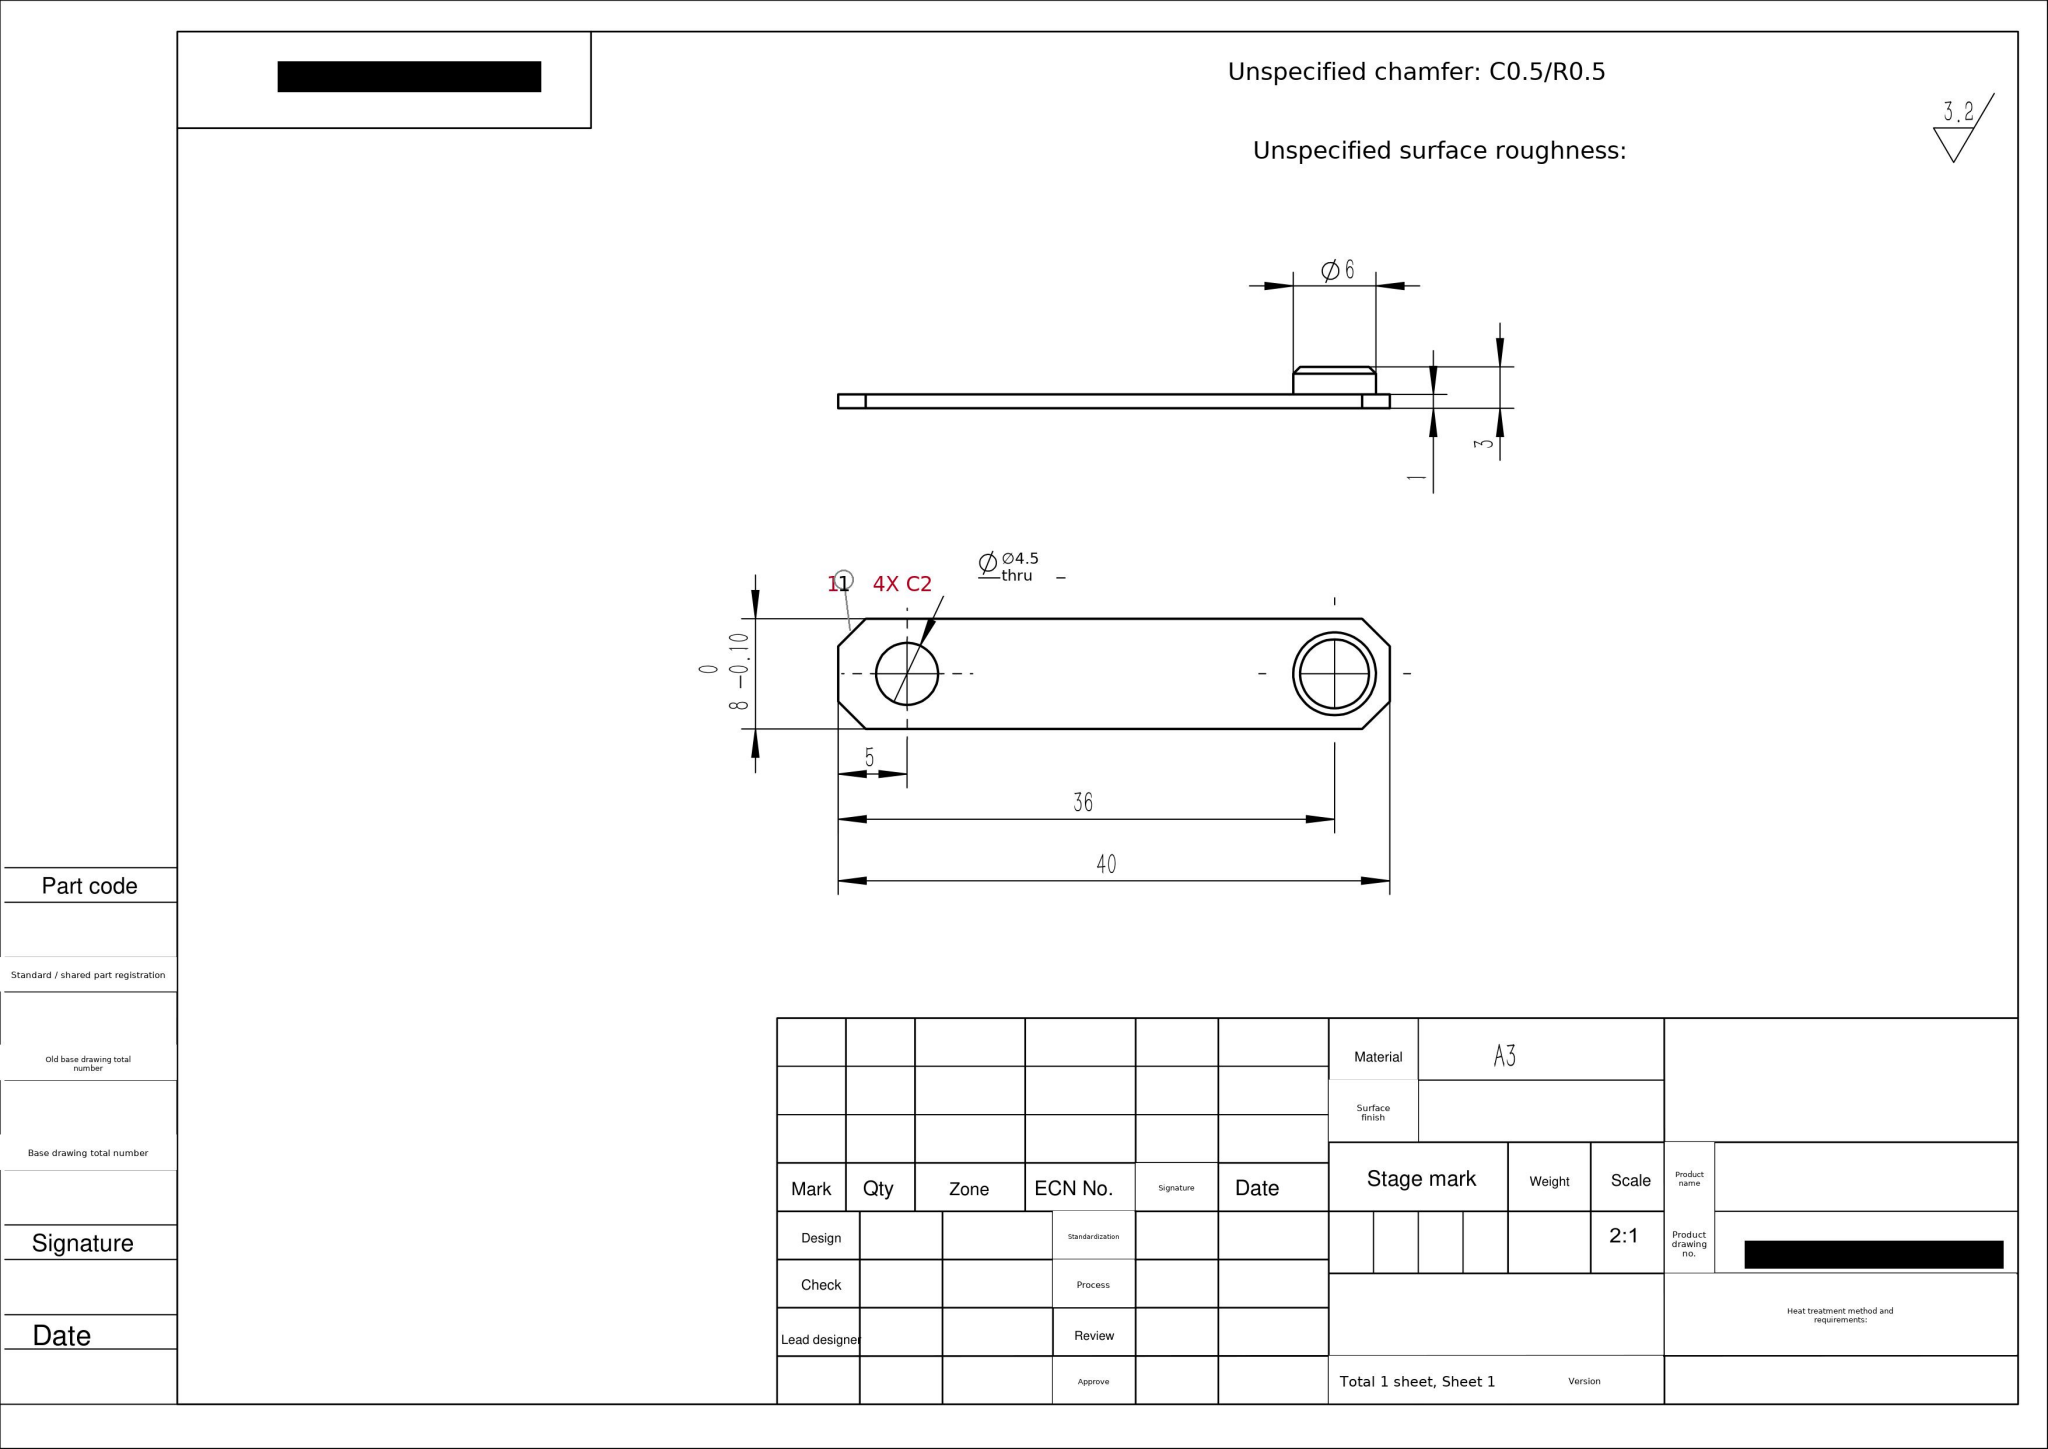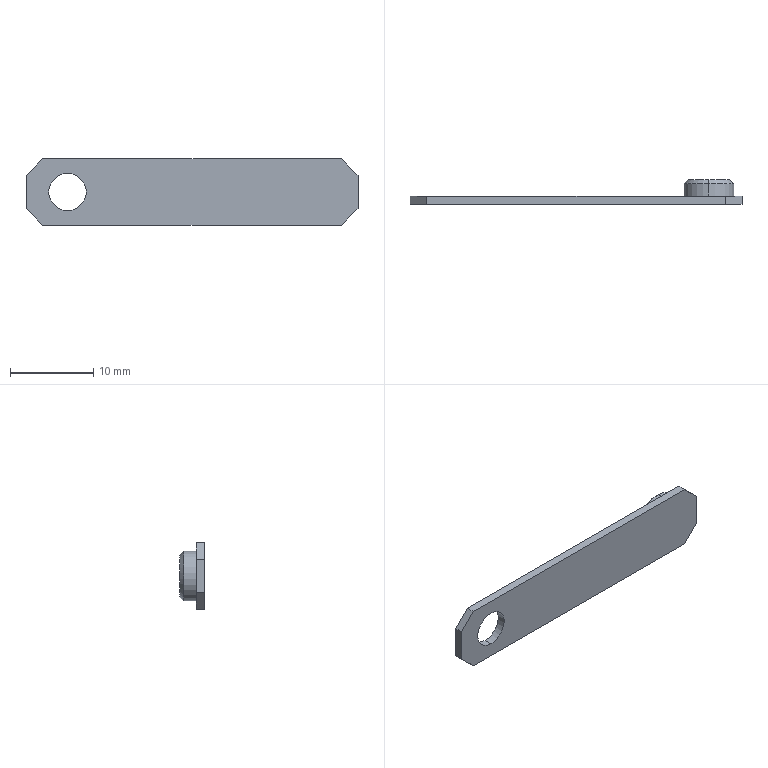Part | SolidWorks | mm | material A3 | 1 solid | 17 faces | box 40 x 3 x 8 mm | volume 350 mm3 | plane 11 | cylinder 4 | cone 2 | commonest cylinder face diameters 4.5 x2 6 x2
build123d program:
from build123d import *

# Parameters (mm, degrees)
SKETCH1_W           = 40
SKETCH1_H           = 8
BOSS_EXTRUDE1_DEPTH = 2
SKETCH2_R           = 2.25
CUT_EXTRUDE1_DEPTH  = 32.281
SKETCH3_R           = 3
BOSS_EXTRUDE2_DEPTH = 1
CHAMFER1_SIZE       = 0.5
CUT_EXTRUDE2_START  = -1
SKETCH4_W           = 49.789
SKETCH4_H           = 17.489
SKETCH4_R           = 3
CUT_EXTRUDE2_DEPTH  = 1
CHAMFER2_SIZE       = 2


with BuildPart() as part:
    # Sketch1 → Boss-Extrude1 (new body)
    with BuildSketch(Plane(origin=(0, 0, 0), x_dir=(1, 0, 0), z_dir=(0, 1, 0))):
        with Locations((10.307, 3.484)):
            Rectangle(SKETCH1_W, SKETCH1_H)
    extrude(amount=BOSS_EXTRUDE1_DEPTH)

    # Sketch2 → Cut-Extrude1 (cut, through all)
    with BuildSketch(Plane(origin=(0, 2, 0), x_dir=(1, 0, 0), z_dir=(0, 1, 0))):
        with Locations(Location((-4.693, 3.484, 0), (0, 0, 270))):
            Circle(SKETCH2_R)
    extrude(amount=-CUT_EXTRUDE1_DEPTH, mode=Mode.SUBTRACT)

    # Sketch3 → Boss-Extrude2 (add)
    with BuildSketch(Plane(origin=(0, 2, 0), x_dir=(1, 0, 0), z_dir=(0, 1, 0))):
        with Locations(Location((26.307, 3.484, 0), (0, 0, 270))):
            Circle(SKETCH3_R)
    extrude(amount=BOSS_EXTRUDE2_DEPTH)

    # Chamfer1
    chamfer1_edges = [part.edges().sort_by_distance(p)[0] for p in [
        (26.307, 3, -6.484),
    ]]
    chamfer(chamfer1_edges, length=CHAMFER1_SIZE)

    # Sketch4 → Cut-Extrude2 (cut)
    with BuildSketch(Plane(origin=(0, 2, 0), x_dir=(1, 0, 0), z_dir=(0, 1, 0)).offset(CUT_EXTRUDE2_START)):
        with Locations((15.201, 2.858)):
            Rectangle(SKETCH4_W, SKETCH4_H)
        with Locations(Location((26.307, 3.484, 0), (0, 0, 270))):
            Circle(SKETCH4_R, mode=Mode.SUBTRACT)
    extrude(amount=CUT_EXTRUDE2_DEPTH, mode=Mode.SUBTRACT)

    # Chamfer2
    chamfer2_edges = [part.edges().sort_by_distance(p)[0] for p in [
        (-9.693, 0.5, -7.484),
        (30.307, 0.5, -7.484),
        (30.307, 0.5, 0.5156),
        (-9.693, 0.5, 0.5156),
    ]]
    chamfer(chamfer2_edges, length=CHAMFER2_SIZE)


solid = part.part
STEP:
#1=CARTESIAN_POINT('',(-4.693,0.,-5.734));
#2=VERTEX_POINT('',#1);
#3=CARTESIAN_POINT('',(-4.693,0.,-1.234));
#4=VERTEX_POINT('',#3);
#5=CARTESIAN_POINT('',(-4.693,0.,-3.484));
#6=DIRECTION('',(0.,1.,0.));
#7=DIRECTION('',(0.,0.,1.));
#8=AXIS2_PLACEMENT_3D('',#5,#6,#7);
#9=CIRCLE('',#8,2.25);
#10=EDGE_CURVE('',#2,#4,#9,.T.);
#11=ORIENTED_EDGE('',*,*,#10,.F.);
#12=CARTESIAN_POINT('',(-4.693,1.,-5.734));
#13=VERTEX_POINT('',#12);
#14=CARTESIAN_POINT('',(-4.693,0.,-5.734));
#15=DIRECTION('',(0.,1.,0.));
#16=VECTOR('',#15,1000.);
#17=LINE('',#14,#16);
#18=EDGE_CURVE('',#2,#13,#17,.T.);
#19=ORIENTED_EDGE('',*,*,#18,.T.);
#20=CARTESIAN_POINT('',(-4.693,1.,-1.234));
#21=VERTEX_POINT('',#20);
#22=CARTESIAN_POINT('',(-4.693,1.,-3.484));
#23=DIRECTION('',(0.,-1.,0.));
#24=DIRECTION('',(0.,0.,1.));
#25=AXIS2_PLACEMENT_3D('',#22,#23,#24);
#26=CIRCLE('',#25,2.25);
#27=EDGE_CURVE('',#21,#13,#26,.T.);
#28=ORIENTED_EDGE('',*,*,#27,.F.);
#29=CARTESIAN_POINT('',(-4.693,0.,-1.234));
#30=DIRECTION('',(0.,1.,0.));
#31=VECTOR('',#30,1000.);
#32=LINE('',#29,#31);
#33=EDGE_CURVE('',#4,#21,#32,.T.);
#34=ORIENTED_EDGE('',*,*,#33,.F.);
#35=EDGE_LOOP('',(#11,#19,#28,#34));
#36=FACE_OUTER_BOUND('',#35,.T.);
#37=CARTESIAN_POINT('',(-4.693,0.,-3.484));
#38=DIRECTION('',(0.,1.,0.));
#39=DIRECTION('',(0.,0.,1.));
#40=AXIS2_PLACEMENT_3D('',#37,#38,#39);
#41=CYLINDRICAL_SURFACE('',#40,2.25);
#42=ADVANCED_FACE('',(#36),#41,.F.);
#43=CARTESIAN_POINT('',(26.307,3.,-0.9844));
#44=VERTEX_POINT('',#43);
#45=CARTESIAN_POINT('',(26.307,3.,-5.984));
#46=VERTEX_POINT('',#45);
#47=CARTESIAN_POINT('',(26.307,3.,-3.484));
#48=DIRECTION('',(0.,1.,0.));
#49=DIRECTION('',(0.,0.,1.));
#50=AXIS2_PLACEMENT_3D('',#47,#48,#49);
#51=CIRCLE('',#50,2.5);
#52=EDGE_CURVE('',#44,#46,#51,.T.);
#53=ORIENTED_EDGE('',*,*,#52,.F.);
#54=CARTESIAN_POINT('',(26.307,2.5,-0.4844));
#55=VERTEX_POINT('',#54);
#56=CARTESIAN_POINT('',(26.307,3.,-0.9844));
#57=DIRECTION('',(0.,-0.7071,0.7071));
#58=VECTOR('',#57,1000.);
#59=LINE('',#56,#58);
#60=EDGE_CURVE('',#44,#55,#59,.T.);
#61=ORIENTED_EDGE('',*,*,#60,.T.);
#62=CARTESIAN_POINT('',(26.307,2.5,-6.484));
#63=VERTEX_POINT('',#62);
#64=CARTESIAN_POINT('',(26.307,2.5,-3.484));
#65=DIRECTION('',(0.,-1.,0.));
#66=DIRECTION('',(0.,0.,1.));
#67=AXIS2_PLACEMENT_3D('',#64,#65,#66);
#68=CIRCLE('',#67,3.);
#69=EDGE_CURVE('',#63,#55,#68,.T.);
#70=ORIENTED_EDGE('',*,*,#69,.F.);
#71=CARTESIAN_POINT('',(26.307,3.,-5.984));
#72=DIRECTION('',(0.,-0.7071,-0.7071));
#73=VECTOR('',#72,1000.);
#74=LINE('',#71,#73);
#75=EDGE_CURVE('',#46,#63,#74,.T.);
#76=ORIENTED_EDGE('',*,*,#75,.F.);
#77=EDGE_LOOP('',(#53,#61,#70,#76));
#78=FACE_OUTER_BOUND('',#77,.T.);
#79=CARTESIAN_POINT('',(26.307,3.,-3.484));
#80=DIRECTION('',(0.,-1.,0.));
#81=DIRECTION('',(0.,0.,-1.));
#82=AXIS2_PLACEMENT_3D('',#79,#80,#81);
#83=CONICAL_SURFACE('',#82,2.5,0.7854);
#84=ADVANCED_FACE('',(#78),#83,.T.);
#85=ORIENTED_EDGE('',*,*,#69,.T.);
#86=CARTESIAN_POINT('',(26.307,1.,-0.4844));
#87=VERTEX_POINT('',#86);
#88=CARTESIAN_POINT('',(26.307,3.,-0.4844));
#89=DIRECTION('',(0.,-1.,0.));
#90=VECTOR('',#89,1000.);
#91=LINE('',#88,#90);
#92=EDGE_CURVE('',#55,#87,#91,.T.);
#93=ORIENTED_EDGE('',*,*,#92,.T.);
#94=CARTESIAN_POINT('',(26.307,1.,-6.484));
#95=VERTEX_POINT('',#94);
#96=CARTESIAN_POINT('',(26.307,1.,-3.484));
#97=DIRECTION('',(0.,1.,0.));
#98=DIRECTION('',(0.,0.,1.));
#99=AXIS2_PLACEMENT_3D('',#96,#97,#98);
#100=CIRCLE('',#99,3.);
#101=EDGE_CURVE('',#87,#95,#100,.T.);
#102=ORIENTED_EDGE('',*,*,#101,.T.);
#103=CARTESIAN_POINT('',(26.307,3.,-6.484));
#104=DIRECTION('',(0.,-1.,0.));
#105=VECTOR('',#104,1000.);
#106=LINE('',#103,#105);
#107=EDGE_CURVE('',#63,#95,#106,.T.);
#108=ORIENTED_EDGE('',*,*,#107,.F.);
#109=EDGE_LOOP('',(#85,#93,#102,#108));
#110=FACE_OUTER_BOUND('',#109,.T.);
#111=CARTESIAN_POINT('',(26.307,3.,-3.484));
#112=DIRECTION('',(0.,-1.,0.));
#113=DIRECTION('',(0.,0.,-1.));
#114=AXIS2_PLACEMENT_3D('',#111,#112,#113);
#115=CYLINDRICAL_SURFACE('',#114,3.);
#116=ADVANCED_FACE('',(#110),#115,.T.);
#117=ORIENTED_EDGE('',*,*,#92,.F.);
#118=CARTESIAN_POINT('',(26.307,2.5,-3.484));
#119=DIRECTION('',(0.,-1.,0.));
#120=DIRECTION('',(0.,0.,1.));
#121=AXIS2_PLACEMENT_3D('',#118,#119,#120);
#122=CIRCLE('',#121,3.);
#123=EDGE_CURVE('',#55,#63,#122,.T.);
#124=ORIENTED_EDGE('',*,*,#123,.T.);
#125=ORIENTED_EDGE('',*,*,#107,.T.);
#126=CARTESIAN_POINT('',(26.307,1.,-3.484));
#127=DIRECTION('',(0.,1.,0.));
#128=DIRECTION('',(0.,0.,1.));
#129=AXIS2_PLACEMENT_3D('',#126,#127,#128);
#130=CIRCLE('',#129,3.);
#131=EDGE_CURVE('',#95,#87,#130,.T.);
#132=ORIENTED_EDGE('',*,*,#131,.T.);
#133=EDGE_LOOP('',(#117,#124,#125,#132));
#134=FACE_OUTER_BOUND('',#133,.T.);
#135=CARTESIAN_POINT('',(26.307,3.,-3.484));
#136=DIRECTION('',(0.,-1.,0.));
#137=DIRECTION('',(0.,0.,-1.));
#138=AXIS2_PLACEMENT_3D('',#135,#136,#137);
#139=CYLINDRICAL_SURFACE('',#138,3.);
#140=ADVANCED_FACE('',(#134),#139,.T.);
#141=CARTESIAN_POINT('',(26.307,3.,-3.484));
#142=DIRECTION('',(0.,1.,0.));
#143=DIRECTION('',(0.,0.,1.));
#144=AXIS2_PLACEMENT_3D('',#141,#142,#143);
#145=CIRCLE('',#144,2.5);
#146=EDGE_CURVE('',#46,#44,#145,.T.);
#147=ORIENTED_EDGE('',*,*,#146,.T.);
#148=ORIENTED_EDGE('',*,*,#52,.T.);
#149=EDGE_LOOP('',(#147,#148));
#150=FACE_OUTER_BOUND('',#149,.T.);
#151=CARTESIAN_POINT('',(26.307,3.,-3.484));
#152=DIRECTION('',(0.,1.,0.));
#153=DIRECTION('',(0.,0.,1.));
#154=AXIS2_PLACEMENT_3D('',#151,#152,#153);
#155=PLANE('',#154);
#156=ADVANCED_FACE('',(#150),#155,.T.);
#157=ORIENTED_EDGE('',*,*,#60,.F.);
#158=ORIENTED_EDGE('',*,*,#146,.F.);
#159=ORIENTED_EDGE('',*,*,#75,.T.);
#160=ORIENTED_EDGE('',*,*,#123,.F.);
#161=EDGE_LOOP('',(#157,#158,#159,#160));
#162=FACE_OUTER_BOUND('',#161,.T.);
#163=CARTESIAN_POINT('',(26.307,3.,-3.484));
#164=DIRECTION('',(0.,-1.,0.));
#165=DIRECTION('',(0.,0.,-1.));
#166=AXIS2_PLACEMENT_3D('',#163,#164,#165);
#167=CONICAL_SURFACE('',#166,2.5,0.7854);
#168=ADVANCED_FACE('',(#162),#167,.T.);
#169=ORIENTED_EDGE('',*,*,#27,.T.);
#170=CARTESIAN_POINT('',(-4.693,1.,-3.484));
#171=DIRECTION('',(0.,-1.,0.));
#172=DIRECTION('',(0.,0.,1.));
#173=AXIS2_PLACEMENT_3D('',#170,#171,#172);
#174=CIRCLE('',#173,2.25);
#175=EDGE_CURVE('',#13,#21,#174,.T.);
#176=ORIENTED_EDGE('',*,*,#175,.T.);
#177=EDGE_LOOP('',(#169,#176));
#178=FACE_BOUND('',#177,.T.);
#179=ORIENTED_EDGE('',*,*,#131,.F.);
#180=ORIENTED_EDGE('',*,*,#101,.F.);
#181=EDGE_LOOP('',(#179,#180));
#182=FACE_BOUND('',#181,.T.);
#183=CARTESIAN_POINT('',(30.307,1.,-1.484));
#184=VERTEX_POINT('',#183);
#185=CARTESIAN_POINT('',(30.307,1.,-5.484));
#186=VERTEX_POINT('',#185);
#187=CARTESIAN_POINT('',(30.307,1.,-7.484));
#188=DIRECTION('',(0.,0.,-1.));
#189=VECTOR('',#188,1000.);
#190=LINE('',#187,#189);
#191=EDGE_CURVE('',#184,#186,#190,.T.);
#192=ORIENTED_EDGE('',*,*,#191,.T.);
#193=CARTESIAN_POINT('',(28.307,1.,-7.484));
#194=VERTEX_POINT('',#193);
#195=CARTESIAN_POINT('',(17.896,1.,-17.896));
#196=DIRECTION('',(-0.7071,0.,-0.7071));
#197=VECTOR('',#196,1000.);
#198=LINE('',#195,#197);
#199=EDGE_CURVE('',#186,#194,#198,.T.);
#200=ORIENTED_EDGE('',*,*,#199,.T.);
#201=CARTESIAN_POINT('',(-7.693,1.,-7.484));
#202=VERTEX_POINT('',#201);
#203=CARTESIAN_POINT('',(-9.693,1.,-7.484));
#204=DIRECTION('',(-1.,0.,0.));
#205=VECTOR('',#204,1000.);
#206=LINE('',#203,#205);
#207=EDGE_CURVE('',#194,#202,#206,.T.);
#208=ORIENTED_EDGE('',*,*,#207,.T.);
#209=CARTESIAN_POINT('',(-9.693,1.,-5.484));
#210=VERTEX_POINT('',#209);
#211=CARTESIAN_POINT('',(-7.589,1.,-7.589));
#212=DIRECTION('',(-0.7071,0.,0.7071));
#213=VECTOR('',#212,1000.);
#214=LINE('',#211,#213);
#215=EDGE_CURVE('',#202,#210,#214,.T.);
#216=ORIENTED_EDGE('',*,*,#215,.T.);
#217=CARTESIAN_POINT('',(-9.693,1.,-1.484));
#218=VERTEX_POINT('',#217);
#219=CARTESIAN_POINT('',(-9.693,1.,-11.603));
#220=DIRECTION('',(0.,0.,1.));
#221=VECTOR('',#220,1000.);
#222=LINE('',#219,#221);
#223=EDGE_CURVE('',#210,#218,#222,.T.);
#224=ORIENTED_EDGE('',*,*,#223,.T.);
#225=CARTESIAN_POINT('',(-7.693,1.,0.5156));
#226=VERTEX_POINT('',#225);
#227=CARTESIAN_POINT('',(-4.104,1.,4.104));
#228=DIRECTION('',(0.7071,0.,0.7071));
#229=VECTOR('',#228,1000.);
#230=LINE('',#227,#229);
#231=EDGE_CURVE('',#218,#226,#230,.T.);
#232=ORIENTED_EDGE('',*,*,#231,.T.);
#233=CARTESIAN_POINT('',(28.307,1.,0.5156));
#234=VERTEX_POINT('',#233);
#235=CARTESIAN_POINT('',(-9.693,1.,0.5156));
#236=DIRECTION('',(1.,0.,0.));
#237=VECTOR('',#236,1000.);
#238=LINE('',#235,#237);
#239=EDGE_CURVE('',#226,#234,#238,.T.);
#240=ORIENTED_EDGE('',*,*,#239,.T.);
#241=CARTESIAN_POINT('',(14.411,1.,14.411));
#242=DIRECTION('',(0.7071,0.,-0.7071));
#243=VECTOR('',#242,1000.);
#244=LINE('',#241,#243);
#245=EDGE_CURVE('',#234,#184,#244,.T.);
#246=ORIENTED_EDGE('',*,*,#245,.T.);
#247=EDGE_LOOP('',(#192,#200,#208,#216,#224,#232,#240,#246));
#248=FACE_OUTER_BOUND('',#247,.T.);
#249=CARTESIAN_POINT('',(0.,1.,0.));
#250=DIRECTION('',(0.,1.,0.));
#251=DIRECTION('',(0.,0.,1.));
#252=AXIS2_PLACEMENT_3D('',#249,#250,#251);
#253=PLANE('',#252);
#254=ADVANCED_FACE('',(#178,#182,#248),#253,.T.);
#255=ORIENTED_EDGE('',*,*,#207,.F.);
#256=CARTESIAN_POINT('',(28.307,0.,-7.484));
#257=VERTEX_POINT('',#256);
#258=CARTESIAN_POINT('',(28.307,2.,-7.484));
#259=DIRECTION('',(0.,-1.,0.));
#260=VECTOR('',#259,1000.);
#261=LINE('',#258,#260);
#262=EDGE_CURVE('',#194,#257,#261,.T.);
#263=ORIENTED_EDGE('',*,*,#262,.T.);
#264=CARTESIAN_POINT('',(-7.693,0.,-7.484));
#265=VERTEX_POINT('',#264);
#266=CARTESIAN_POINT('',(-9.693,0.,-7.484));
#267=DIRECTION('',(-1.,0.,0.));
#268=VECTOR('',#267,1000.);
#269=LINE('',#266,#268);
#270=EDGE_CURVE('',#257,#265,#269,.T.);
#271=ORIENTED_EDGE('',*,*,#270,.T.);
#272=CARTESIAN_POINT('',(-7.693,2.,-7.484));
#273=DIRECTION('',(0.,1.,0.));
#274=VECTOR('',#273,1000.);
#275=LINE('',#272,#274);
#276=EDGE_CURVE('',#265,#202,#275,.T.);
#277=ORIENTED_EDGE('',*,*,#276,.T.);
#278=EDGE_LOOP('',(#255,#263,#271,#277));
#279=FACE_OUTER_BOUND('',#278,.T.);
#280=CARTESIAN_POINT('',(-9.693,2.,-7.484));
#281=DIRECTION('',(0.,0.,1.));
#282=DIRECTION('',(1.,0.,0.));
#283=AXIS2_PLACEMENT_3D('',#280,#281,#282);
#284=PLANE('',#283);
#285=ADVANCED_FACE('',(#279),#284,.F.);
#286=CARTESIAN_POINT('',(30.307,0.,-1.484));
#287=VERTEX_POINT('',#286);
#288=CARTESIAN_POINT('',(30.307,0.,-5.484));
#289=VERTEX_POINT('',#288);
#290=CARTESIAN_POINT('',(30.307,0.,-7.484));
#291=DIRECTION('',(0.,0.,-1.));
#292=VECTOR('',#291,1000.);
#293=LINE('',#290,#292);
#294=EDGE_CURVE('',#287,#289,#293,.T.);
#295=ORIENTED_EDGE('',*,*,#294,.T.);
#296=CARTESIAN_POINT('',(30.307,2.,-5.484));
#297=DIRECTION('',(0.,1.,0.));
#298=VECTOR('',#297,1000.);
#299=LINE('',#296,#298);
#300=EDGE_CURVE('',#289,#186,#299,.T.);
#301=ORIENTED_EDGE('',*,*,#300,.T.);
#302=ORIENTED_EDGE('',*,*,#191,.F.);
#303=CARTESIAN_POINT('',(30.307,2.,-1.484));
#304=DIRECTION('',(0.,-1.,0.));
#305=VECTOR('',#304,1000.);
#306=LINE('',#303,#305);
#307=EDGE_CURVE('',#184,#287,#306,.T.);
#308=ORIENTED_EDGE('',*,*,#307,.T.);
#309=EDGE_LOOP('',(#295,#301,#302,#308));
#310=FACE_OUTER_BOUND('',#309,.T.);
#311=CARTESIAN_POINT('',(30.307,2.,-7.484));
#312=DIRECTION('',(-1.,0.,0.));
#313=DIRECTION('',(0.,0.,1.));
#314=AXIS2_PLACEMENT_3D('',#311,#312,#313);
#315=PLANE('',#314);
#316=ADVANCED_FACE('',(#310),#315,.F.);
#317=CARTESIAN_POINT('',(-7.693,0.,0.5156));
#318=VERTEX_POINT('',#317);
#319=CARTESIAN_POINT('',(28.307,0.,0.5156));
#320=VERTEX_POINT('',#319);
#321=CARTESIAN_POINT('',(-9.693,0.,0.5156));
#322=DIRECTION('',(1.,0.,0.));
#323=VECTOR('',#322,1000.);
#324=LINE('',#321,#323);
#325=EDGE_CURVE('',#318,#320,#324,.T.);
#326=ORIENTED_EDGE('',*,*,#325,.T.);
#327=CARTESIAN_POINT('',(28.307,2.,0.5156));
#328=DIRECTION('',(0.,1.,0.));
#329=VECTOR('',#328,1000.);
#330=LINE('',#327,#329);
#331=EDGE_CURVE('',#320,#234,#330,.T.);
#332=ORIENTED_EDGE('',*,*,#331,.T.);
#333=ORIENTED_EDGE('',*,*,#239,.F.);
#334=CARTESIAN_POINT('',(-7.693,2.,0.5156));
#335=DIRECTION('',(0.,-1.,0.));
#336=VECTOR('',#335,1000.);
#337=LINE('',#334,#336);
#338=EDGE_CURVE('',#226,#318,#337,.T.);
#339=ORIENTED_EDGE('',*,*,#338,.T.);
#340=EDGE_LOOP('',(#326,#332,#333,#339));
#341=FACE_OUTER_BOUND('',#340,.T.);
#342=CARTESIAN_POINT('',(-9.693,2.,0.5156));
#343=DIRECTION('',(0.,0.,-1.));
#344=DIRECTION('',(-1.,0.,-0.));
#345=AXIS2_PLACEMENT_3D('',#342,#343,#344);
#346=PLANE('',#345);
#347=ADVANCED_FACE('',(#341),#346,.F.);
#348=CARTESIAN_POINT('',(-9.693,0.,-5.484));
#349=VERTEX_POINT('',#348);
#350=CARTESIAN_POINT('',(-9.693,0.,-1.484));
#351=VERTEX_POINT('',#350);
#352=CARTESIAN_POINT('',(-9.693,0.,-7.484));
#353=DIRECTION('',(0.,0.,1.));
#354=VECTOR('',#353,1000.);
#355=LINE('',#352,#354);
#356=EDGE_CURVE('',#349,#351,#355,.T.);
#357=ORIENTED_EDGE('',*,*,#356,.T.);
#358=CARTESIAN_POINT('',(-9.693,2.,-1.484));
#359=DIRECTION('',(0.,1.,0.));
#360=VECTOR('',#359,1000.);
#361=LINE('',#358,#360);
#362=EDGE_CURVE('',#351,#218,#361,.T.);
#363=ORIENTED_EDGE('',*,*,#362,.T.);
#364=ORIENTED_EDGE('',*,*,#223,.F.);
#365=CARTESIAN_POINT('',(-9.693,2.,-5.484));
#366=DIRECTION('',(0.,-1.,0.));
#367=VECTOR('',#366,1000.);
#368=LINE('',#365,#367);
#369=EDGE_CURVE('',#210,#349,#368,.T.);
#370=ORIENTED_EDGE('',*,*,#369,.T.);
#371=EDGE_LOOP('',(#357,#363,#364,#370));
#372=FACE_OUTER_BOUND('',#371,.T.);
#373=CARTESIAN_POINT('',(-9.693,2.,-7.484));
#374=DIRECTION('',(1.,0.,0.));
#375=DIRECTION('',(0.,0.,-1.));
#376=AXIS2_PLACEMENT_3D('',#373,#374,#375);
#377=PLANE('',#376);
#378=ADVANCED_FACE('',(#372),#377,.F.);
#379=CARTESIAN_POINT('',(-4.693,0.,-3.484));
#380=DIRECTION('',(0.,1.,0.));
#381=DIRECTION('',(0.,0.,1.));
#382=AXIS2_PLACEMENT_3D('',#379,#380,#381);
#383=CIRCLE('',#382,2.25);
#384=EDGE_CURVE('',#4,#2,#383,.T.);
#385=ORIENTED_EDGE('',*,*,#384,.T.);
#386=ORIENTED_EDGE('',*,*,#10,.T.);
#387=EDGE_LOOP('',(#385,#386));
#388=FACE_BOUND('',#387,.T.);
#389=ORIENTED_EDGE('',*,*,#270,.F.);
#390=CARTESIAN_POINT('',(28.307,0.,-7.484));
#391=DIRECTION('',(0.7071,0.,0.7071));
#392=VECTOR('',#391,1000.);
#393=LINE('',#390,#392);
#394=EDGE_CURVE('',#257,#289,#393,.T.);
#395=ORIENTED_EDGE('',*,*,#394,.T.);
#396=ORIENTED_EDGE('',*,*,#294,.F.);
#397=CARTESIAN_POINT('',(30.307,0.,-1.484));
#398=DIRECTION('',(-0.7071,0.,0.7071));
#399=VECTOR('',#398,1000.);
#400=LINE('',#397,#399);
#401=EDGE_CURVE('',#287,#320,#400,.T.);
#402=ORIENTED_EDGE('',*,*,#401,.T.);
#403=ORIENTED_EDGE('',*,*,#325,.F.);
#404=CARTESIAN_POINT('',(-7.693,0.,0.5156));
#405=DIRECTION('',(-0.7071,0.,-0.7071));
#406=VECTOR('',#405,1000.);
#407=LINE('',#404,#406);
#408=EDGE_CURVE('',#318,#351,#407,.T.);
#409=ORIENTED_EDGE('',*,*,#408,.T.);
#410=ORIENTED_EDGE('',*,*,#356,.F.);
#411=CARTESIAN_POINT('',(-9.693,0.,-5.484));
#412=DIRECTION('',(0.7071,0.,-0.7071));
#413=VECTOR('',#412,1000.);
#414=LINE('',#411,#413);
#415=EDGE_CURVE('',#349,#265,#414,.T.);
#416=ORIENTED_EDGE('',*,*,#415,.T.);
#417=EDGE_LOOP('',(#389,#395,#396,#402,#403,#409,#410,#416));
#418=FACE_OUTER_BOUND('',#417,.T.);
#419=CARTESIAN_POINT('',(0.,0.,0.));
#420=DIRECTION('',(0.,1.,0.));
#421=DIRECTION('',(0.,0.,1.));
#422=AXIS2_PLACEMENT_3D('',#419,#420,#421);
#423=PLANE('',#422);
#424=ADVANCED_FACE('',(#388,#418),#423,.F.);
#425=ORIENTED_EDGE('',*,*,#18,.F.);
#426=ORIENTED_EDGE('',*,*,#384,.F.);
#427=ORIENTED_EDGE('',*,*,#33,.T.);
#428=ORIENTED_EDGE('',*,*,#175,.F.);
#429=EDGE_LOOP('',(#425,#426,#427,#428));
#430=FACE_OUTER_BOUND('',#429,.T.);
#431=CARTESIAN_POINT('',(-4.693,0.,-3.484));
#432=DIRECTION('',(0.,1.,0.));
#433=DIRECTION('',(0.,0.,1.));
#434=AXIS2_PLACEMENT_3D('',#431,#432,#433);
#435=CYLINDRICAL_SURFACE('',#434,2.25);
#436=ADVANCED_FACE('',(#430),#435,.F.);
#437=ORIENTED_EDGE('',*,*,#199,.F.);
#438=ORIENTED_EDGE('',*,*,#300,.F.);
#439=ORIENTED_EDGE('',*,*,#394,.F.);
#440=ORIENTED_EDGE('',*,*,#262,.F.);
#441=EDGE_LOOP('',(#437,#438,#439,#440));
#442=FACE_OUTER_BOUND('',#441,.T.);
#443=CARTESIAN_POINT('',(28.307,2.,-7.484));
#444=DIRECTION('',(-0.7071,0.,0.7071));
#445=DIRECTION('',(0.,-1.,0.));
#446=AXIS2_PLACEMENT_3D('',#443,#444,#445);
#447=PLANE('',#446);
#448=ADVANCED_FACE('',(#442),#447,.F.);
#449=ORIENTED_EDGE('',*,*,#245,.F.);
#450=ORIENTED_EDGE('',*,*,#331,.F.);
#451=ORIENTED_EDGE('',*,*,#401,.F.);
#452=ORIENTED_EDGE('',*,*,#307,.F.);
#453=EDGE_LOOP('',(#449,#450,#451,#452));
#454=FACE_OUTER_BOUND('',#453,.T.);
#455=CARTESIAN_POINT('',(30.307,2.,-1.484));
#456=DIRECTION('',(-0.7071,0.,-0.7071));
#457=DIRECTION('',(0.,-1.,0.));
#458=AXIS2_PLACEMENT_3D('',#455,#456,#457);
#459=PLANE('',#458);
#460=ADVANCED_FACE('',(#454),#459,.F.);
#461=ORIENTED_EDGE('',*,*,#231,.F.);
#462=ORIENTED_EDGE('',*,*,#362,.F.);
#463=ORIENTED_EDGE('',*,*,#408,.F.);
#464=ORIENTED_EDGE('',*,*,#338,.F.);
#465=EDGE_LOOP('',(#461,#462,#463,#464));
#466=FACE_OUTER_BOUND('',#465,.T.);
#467=CARTESIAN_POINT('',(-7.693,2.,0.5156));
#468=DIRECTION('',(0.7071,0.,-0.7071));
#469=DIRECTION('',(0.,-1.,0.));
#470=AXIS2_PLACEMENT_3D('',#467,#468,#469);
#471=PLANE('',#470);
#472=ADVANCED_FACE('',(#466),#471,.F.);
#473=ORIENTED_EDGE('',*,*,#215,.F.);
#474=ORIENTED_EDGE('',*,*,#276,.F.);
#475=ORIENTED_EDGE('',*,*,#415,.F.);
#476=ORIENTED_EDGE('',*,*,#369,.F.);
#477=EDGE_LOOP('',(#473,#474,#475,#476));
#478=FACE_OUTER_BOUND('',#477,.T.);
#479=CARTESIAN_POINT('',(-9.693,2.,-5.484));
#480=DIRECTION('',(0.7071,0.,0.7071));
#481=DIRECTION('',(0.,-1.,0.));
#482=AXIS2_PLACEMENT_3D('',#479,#480,#481);
#483=PLANE('',#482);
#484=ADVANCED_FACE('',(#478),#483,.F.);
#485=CLOSED_SHELL('',(#42,#84,#116,#140,#156,#168,#254,#285,#316,#347,#378,#424,#436,#448,#460,#472,#484));
#486=MANIFOLD_SOLID_BREP('',#485);
#487=CARTESIAN_POINT('',(0.,0.,0.));
#488=DIRECTION('',(0.,0.,1.));
#489=DIRECTION('',(1.,0.,0.));
#490=AXIS2_PLACEMENT_3D('',#487,#488,#489);
#491=(LENGTH_UNIT()NAMED_UNIT(*)SI_UNIT(.MILLI.,.METRE.));
#492=UNCERTAINTY_MEASURE_WITH_UNIT(LENGTH_MEASURE(0.00001),#491,'','');
#493=(NAMED_UNIT(*)PLANE_ANGLE_UNIT()SI_UNIT($,.RADIAN.));
#494=(NAMED_UNIT(*)SI_UNIT($,.STERADIAN.)SOLID_ANGLE_UNIT());
#495=(GEOMETRIC_REPRESENTATION_CONTEXT(3)GLOBAL_UNCERTAINTY_ASSIGNED_CONTEXT((#492))GLOBAL_UNIT_ASSIGNED_CONTEXT((#491,#493,#494))REPRESENTATION_CONTEXT('',''));
#496=ADVANCED_BREP_SHAPE_REPRESENTATION('',(#486,#490),#495);